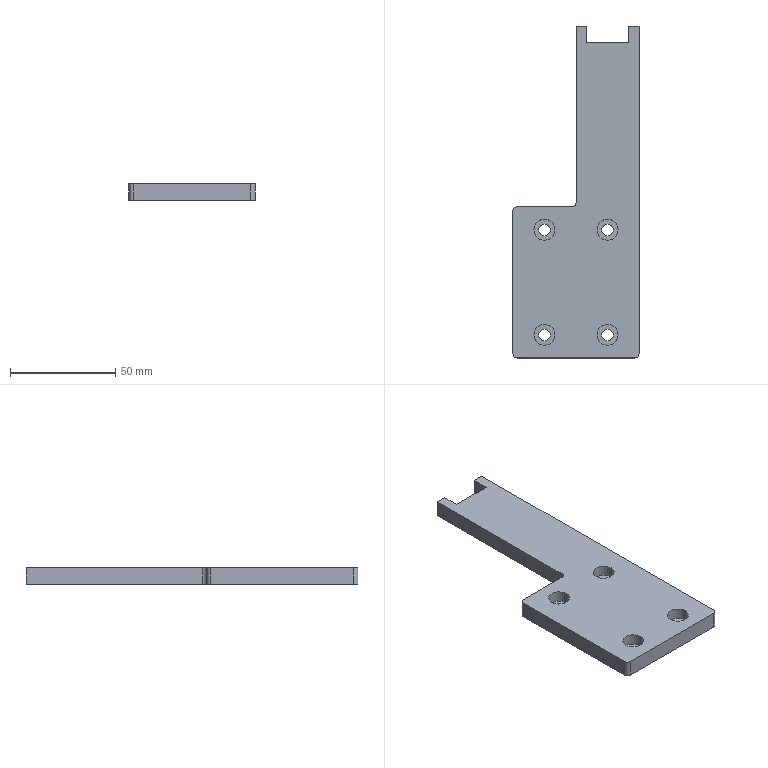Component | SolidWorks | BearingLiftingModule-1_CHEN123-AA-23-1 | 1 solid | 36 faces | box 60 x 158 x 8 mm | volume 51963 mm3 | cylinder 20 | plane 16 | commonest cylinder face diameters 10 x8 5.5 x8 4 x4
build123d program:
from build123d import *

# Parameters (mm, degrees)
SKETCH1_W                                       = 60
SKETCH1_H                                       = 158
BOSS_EXTRUDE1_DEPTH                             = 8
SKETCH2_W                                       = 30
SKETCH2_H                                       = 86
CUT_EXTRUDE1_DEPTH                              = 85.882
SKETCH3_W                                       = 20
SKETCH3_H                                       = 16
CUT_EXTRUDE2_DEPTH                              = 10
FILLET1_R                                       = 2
M5_HEX_SOCKET_HEAD_CAP_SCREW_CBORE1_D           = 5.5
M5_HEX_SOCKET_HEAD_CAP_SCREW_CBORE1_CBORE_D     = 10
M5_HEX_SOCKET_HEAD_CAP_SCREW_CBORE1_CBORE_DEPTH = 5.4


with BuildPart() as part:
    # Sketch1 → Boss-Extrude1 (new body)
    with BuildSketch(Plane.XY):
        Rectangle(SKETCH1_W, SKETCH1_H)
    extrude(amount=BOSS_EXTRUDE1_DEPTH)

    # Sketch2 → Cut-Extrude1 (cut, through all)
    with BuildSketch(Plane.XY.offset(8)):
        with Locations((-15, 36)):
            Rectangle(SKETCH2_W, SKETCH2_H)
    extrude(amount=-CUT_EXTRUDE1_DEPTH, mode=Mode.SUBTRACT)

    # Sketch3 → Cut-Extrude2 (cut)
    with BuildSketch(Plane.XY.offset(8)):
        with Locations((15, 79)):
            Rectangle(SKETCH3_W, SKETCH3_H)
    extrude(amount=-CUT_EXTRUDE2_DEPTH, mode=Mode.SUBTRACT)

    # Fillet1
    fillet1_edges = [part.edges().sort_by_distance(p)[0] for p in [
        (-30, -7, 4),
        (0, -7, 4),
        (30, -79, 4),
        (-30, -79, 4),
    ]]
    fillet(fillet1_edges, radius=FILLET1_R)

    # M5 Hex Socket Head Cap Screw CBORE1 (through all)
    with Locations(Plane.XY.offset(8)):
        with Locations((-15, -18), (15, -18), (-15, -68), (15, -68)):
            CounterBoreHole(M5_HEX_SOCKET_HEAD_CAP_SCREW_CBORE1_D / 2, M5_HEX_SOCKET_HEAD_CAP_SCREW_CBORE1_CBORE_D / 2, M5_HEX_SOCKET_HEAD_CAP_SCREW_CBORE1_CBORE_DEPTH)


solid = part.part

# Placed as in the assembly
solid = solid.moved(Location((54.999, -35.499, 102), (0, 0, 0)))
STEP:
#1=COLOUR_RGB('',0.7922,0.8196,0.9333);
#2=FILL_AREA_STYLE_COLOUR('',#1);
#3=FILL_AREA_STYLE('',(#2));
#4=SURFACE_STYLE_FILL_AREA(#3);
#5=SURFACE_SIDE_STYLE('',(#4));
#6=SURFACE_STYLE_USAGE(.BOTH.,#5);
#7=PRESENTATION_STYLE_ASSIGNMENT((#6));
#8=CARTESIAN_POINT('',(1.378,-2.106,4.118));
#9=VERTEX_POINT('',#8);
#10=CARTESIAN_POINT('',(1.772,-2.106,4.118));
#11=VERTEX_POINT('',#10);
#12=CARTESIAN_POINT('',(1.575,-2.106,4.118));
#13=DIRECTION('',(0.,0.,1.));
#14=DIRECTION('',(1.,0.,0.));
#15=AXIS2_PLACEMENT_3D('',#12,#13,#14);
#16=CIRCLE('',#15,0.1969);
#17=EDGE_CURVE('',#9,#11,#16,.T.);
#18=ORIENTED_EDGE('',*,*,#17,.F.);
#19=CARTESIAN_POINT('',(1.378,-2.106,4.331));
#20=VERTEX_POINT('',#19);
#21=CARTESIAN_POINT('',(1.378,-2.106,4.331));
#22=DIRECTION('',(0.,0.,1.));
#23=VECTOR('',#22,39.37);
#24=LINE('',#21,#23);
#25=EDGE_CURVE('',#9,#20,#24,.T.);
#26=ORIENTED_EDGE('',*,*,#25,.T.);
#27=CARTESIAN_POINT('',(1.772,-2.106,4.331));
#28=VERTEX_POINT('',#27);
#29=CARTESIAN_POINT('',(1.575,-2.106,4.331));
#30=DIRECTION('',(0.,0.,1.));
#31=DIRECTION('',(1.,0.,0.));
#32=AXIS2_PLACEMENT_3D('',#29,#30,#31);
#33=CIRCLE('',#32,0.1969);
#34=EDGE_CURVE('',#20,#28,#33,.T.);
#35=ORIENTED_EDGE('',*,*,#34,.T.);
#36=CARTESIAN_POINT('',(1.772,-2.106,4.331));
#37=DIRECTION('',(0.,0.,1.));
#38=VECTOR('',#37,39.37);
#39=LINE('',#36,#38);
#40=EDGE_CURVE('',#11,#28,#39,.T.);
#41=ORIENTED_EDGE('',*,*,#40,.F.);
#42=EDGE_LOOP('',(#18,#26,#35,#41));
#43=FACE_OUTER_BOUND('',#42,.T.);
#44=CARTESIAN_POINT('',(1.575,-2.106,4.331));
#45=DIRECTION('',(0.,0.,1.));
#46=DIRECTION('',(1.,0.,0.));
#47=AXIS2_PLACEMENT_3D('',#44,#45,#46);
#48=CYLINDRICAL_SURFACE('',#47,0.1969);
#49=ADVANCED_FACE('',(#43),#48,.F.);
#50=CARTESIAN_POINT('',(1.467,-2.106,4.016));
#51=VERTEX_POINT('',#50);
#52=CARTESIAN_POINT('',(1.683,-2.106,4.016));
#53=VERTEX_POINT('',#52);
#54=CARTESIAN_POINT('',(1.575,-2.106,4.016));
#55=DIRECTION('',(0.,0.,1.));
#56=DIRECTION('',(1.,0.,0.));
#57=AXIS2_PLACEMENT_3D('',#54,#55,#56);
#58=CIRCLE('',#57,0.1083);
#59=EDGE_CURVE('',#51,#53,#58,.T.);
#60=ORIENTED_EDGE('',*,*,#59,.F.);
#61=CARTESIAN_POINT('',(1.467,-2.106,4.118));
#62=VERTEX_POINT('',#61);
#63=CARTESIAN_POINT('',(1.467,-2.106,4.331));
#64=DIRECTION('',(0.,0.,1.));
#65=VECTOR('',#64,39.37);
#66=LINE('',#63,#65);
#67=EDGE_CURVE('',#51,#62,#66,.T.);
#68=ORIENTED_EDGE('',*,*,#67,.T.);
#69=CARTESIAN_POINT('',(1.683,-2.106,4.118));
#70=VERTEX_POINT('',#69);
#71=CARTESIAN_POINT('',(1.575,-2.106,4.118));
#72=DIRECTION('',(0.,0.,1.));
#73=DIRECTION('',(1.,0.,0.));
#74=AXIS2_PLACEMENT_3D('',#71,#72,#73);
#75=CIRCLE('',#74,0.1083);
#76=EDGE_CURVE('',#62,#70,#75,.T.);
#77=ORIENTED_EDGE('',*,*,#76,.T.);
#78=CARTESIAN_POINT('',(1.683,-2.106,4.331));
#79=DIRECTION('',(0.,0.,1.));
#80=VECTOR('',#79,39.37);
#81=LINE('',#78,#80);
#82=EDGE_CURVE('',#53,#70,#81,.T.);
#83=ORIENTED_EDGE('',*,*,#82,.F.);
#84=EDGE_LOOP('',(#60,#68,#77,#83));
#85=FACE_OUTER_BOUND('',#84,.T.);
#86=CARTESIAN_POINT('',(1.575,-2.106,4.331));
#87=DIRECTION('',(0.,0.,1.));
#88=DIRECTION('',(1.,0.,0.));
#89=AXIS2_PLACEMENT_3D('',#86,#87,#88);
#90=CYLINDRICAL_SURFACE('',#89,0.1083);
#91=ADVANCED_FACE('',(#85),#90,.F.);
#92=CARTESIAN_POINT('',(2.559,-2.106,4.118));
#93=VERTEX_POINT('',#92);
#94=CARTESIAN_POINT('',(2.953,-2.106,4.118));
#95=VERTEX_POINT('',#94);
#96=CARTESIAN_POINT('',(2.756,-2.106,4.118));
#97=DIRECTION('',(0.,0.,1.));
#98=DIRECTION('',(1.,0.,0.));
#99=AXIS2_PLACEMENT_3D('',#96,#97,#98);
#100=CIRCLE('',#99,0.1969);
#101=EDGE_CURVE('',#93,#95,#100,.T.);
#102=ORIENTED_EDGE('',*,*,#101,.F.);
#103=CARTESIAN_POINT('',(2.559,-2.106,4.331));
#104=VERTEX_POINT('',#103);
#105=CARTESIAN_POINT('',(2.559,-2.106,4.331));
#106=DIRECTION('',(0.,0.,1.));
#107=VECTOR('',#106,39.37);
#108=LINE('',#105,#107);
#109=EDGE_CURVE('',#93,#104,#108,.T.);
#110=ORIENTED_EDGE('',*,*,#109,.T.);
#111=CARTESIAN_POINT('',(2.953,-2.106,4.331));
#112=VERTEX_POINT('',#111);
#113=CARTESIAN_POINT('',(2.756,-2.106,4.331));
#114=DIRECTION('',(0.,0.,1.));
#115=DIRECTION('',(1.,0.,0.));
#116=AXIS2_PLACEMENT_3D('',#113,#114,#115);
#117=CIRCLE('',#116,0.1969);
#118=EDGE_CURVE('',#104,#112,#117,.T.);
#119=ORIENTED_EDGE('',*,*,#118,.T.);
#120=CARTESIAN_POINT('',(2.953,-2.106,4.331));
#121=DIRECTION('',(0.,0.,1.));
#122=VECTOR('',#121,39.37);
#123=LINE('',#120,#122);
#124=EDGE_CURVE('',#95,#112,#123,.T.);
#125=ORIENTED_EDGE('',*,*,#124,.F.);
#126=EDGE_LOOP('',(#102,#110,#119,#125));
#127=FACE_OUTER_BOUND('',#126,.T.);
#128=CARTESIAN_POINT('',(2.756,-2.106,4.331));
#129=DIRECTION('',(0.,0.,1.));
#130=DIRECTION('',(1.,0.,0.));
#131=AXIS2_PLACEMENT_3D('',#128,#129,#130);
#132=CYLINDRICAL_SURFACE('',#131,0.1969);
#133=ADVANCED_FACE('',(#127),#132,.F.);
#134=CARTESIAN_POINT('',(2.648,-2.106,4.016));
#135=VERTEX_POINT('',#134);
#136=CARTESIAN_POINT('',(2.864,-2.106,4.016));
#137=VERTEX_POINT('',#136);
#138=CARTESIAN_POINT('',(2.756,-2.106,4.016));
#139=DIRECTION('',(0.,0.,1.));
#140=DIRECTION('',(1.,0.,0.));
#141=AXIS2_PLACEMENT_3D('',#138,#139,#140);
#142=CIRCLE('',#141,0.1083);
#143=EDGE_CURVE('',#135,#137,#142,.T.);
#144=ORIENTED_EDGE('',*,*,#143,.F.);
#145=CARTESIAN_POINT('',(2.648,-2.106,4.118));
#146=VERTEX_POINT('',#145);
#147=CARTESIAN_POINT('',(2.648,-2.106,4.331));
#148=DIRECTION('',(0.,0.,1.));
#149=VECTOR('',#148,39.37);
#150=LINE('',#147,#149);
#151=EDGE_CURVE('',#135,#146,#150,.T.);
#152=ORIENTED_EDGE('',*,*,#151,.T.);
#153=CARTESIAN_POINT('',(2.864,-2.106,4.118));
#154=VERTEX_POINT('',#153);
#155=CARTESIAN_POINT('',(2.756,-2.106,4.118));
#156=DIRECTION('',(0.,0.,1.));
#157=DIRECTION('',(1.,0.,0.));
#158=AXIS2_PLACEMENT_3D('',#155,#156,#157);
#159=CIRCLE('',#158,0.1083);
#160=EDGE_CURVE('',#146,#154,#159,.T.);
#161=ORIENTED_EDGE('',*,*,#160,.T.);
#162=CARTESIAN_POINT('',(2.864,-2.106,4.331));
#163=DIRECTION('',(0.,0.,1.));
#164=VECTOR('',#163,39.37);
#165=LINE('',#162,#164);
#166=EDGE_CURVE('',#137,#154,#165,.T.);
#167=ORIENTED_EDGE('',*,*,#166,.F.);
#168=EDGE_LOOP('',(#144,#152,#161,#167));
#169=FACE_OUTER_BOUND('',#168,.T.);
#170=CARTESIAN_POINT('',(2.756,-2.106,4.331));
#171=DIRECTION('',(0.,0.,1.));
#172=DIRECTION('',(1.,0.,0.));
#173=AXIS2_PLACEMENT_3D('',#170,#171,#172);
#174=CYLINDRICAL_SURFACE('',#173,0.1083);
#175=ADVANCED_FACE('',(#169),#174,.F.);
#176=CARTESIAN_POINT('',(1.378,-4.075,4.118));
#177=VERTEX_POINT('',#176);
#178=CARTESIAN_POINT('',(1.772,-4.075,4.118));
#179=VERTEX_POINT('',#178);
#180=CARTESIAN_POINT('',(1.575,-4.075,4.118));
#181=DIRECTION('',(0.,0.,1.));
#182=DIRECTION('',(1.,0.,0.));
#183=AXIS2_PLACEMENT_3D('',#180,#181,#182);
#184=CIRCLE('',#183,0.1969);
#185=EDGE_CURVE('',#177,#179,#184,.T.);
#186=ORIENTED_EDGE('',*,*,#185,.F.);
#187=CARTESIAN_POINT('',(1.378,-4.075,4.331));
#188=VERTEX_POINT('',#187);
#189=CARTESIAN_POINT('',(1.378,-4.075,4.331));
#190=DIRECTION('',(0.,0.,1.));
#191=VECTOR('',#190,39.37);
#192=LINE('',#189,#191);
#193=EDGE_CURVE('',#177,#188,#192,.T.);
#194=ORIENTED_EDGE('',*,*,#193,.T.);
#195=CARTESIAN_POINT('',(1.772,-4.075,4.331));
#196=VERTEX_POINT('',#195);
#197=CARTESIAN_POINT('',(1.575,-4.075,4.331));
#198=DIRECTION('',(0.,0.,1.));
#199=DIRECTION('',(1.,0.,0.));
#200=AXIS2_PLACEMENT_3D('',#197,#198,#199);
#201=CIRCLE('',#200,0.1969);
#202=EDGE_CURVE('',#188,#196,#201,.T.);
#203=ORIENTED_EDGE('',*,*,#202,.T.);
#204=CARTESIAN_POINT('',(1.772,-4.075,4.331));
#205=DIRECTION('',(0.,0.,1.));
#206=VECTOR('',#205,39.37);
#207=LINE('',#204,#206);
#208=EDGE_CURVE('',#179,#196,#207,.T.);
#209=ORIENTED_EDGE('',*,*,#208,.F.);
#210=EDGE_LOOP('',(#186,#194,#203,#209));
#211=FACE_OUTER_BOUND('',#210,.T.);
#212=CARTESIAN_POINT('',(1.575,-4.075,4.331));
#213=DIRECTION('',(0.,0.,1.));
#214=DIRECTION('',(1.,0.,0.));
#215=AXIS2_PLACEMENT_3D('',#212,#213,#214);
#216=CYLINDRICAL_SURFACE('',#215,0.1969);
#217=ADVANCED_FACE('',(#211),#216,.F.);
#218=CARTESIAN_POINT('',(1.467,-4.075,4.016));
#219=VERTEX_POINT('',#218);
#220=CARTESIAN_POINT('',(1.683,-4.075,4.016));
#221=VERTEX_POINT('',#220);
#222=CARTESIAN_POINT('',(1.575,-4.075,4.016));
#223=DIRECTION('',(0.,0.,1.));
#224=DIRECTION('',(1.,0.,0.));
#225=AXIS2_PLACEMENT_3D('',#222,#223,#224);
#226=CIRCLE('',#225,0.1083);
#227=EDGE_CURVE('',#219,#221,#226,.T.);
#228=ORIENTED_EDGE('',*,*,#227,.F.);
#229=CARTESIAN_POINT('',(1.467,-4.075,4.118));
#230=VERTEX_POINT('',#229);
#231=CARTESIAN_POINT('',(1.467,-4.075,4.331));
#232=DIRECTION('',(0.,0.,1.));
#233=VECTOR('',#232,39.37);
#234=LINE('',#231,#233);
#235=EDGE_CURVE('',#219,#230,#234,.T.);
#236=ORIENTED_EDGE('',*,*,#235,.T.);
#237=CARTESIAN_POINT('',(1.683,-4.075,4.118));
#238=VERTEX_POINT('',#237);
#239=CARTESIAN_POINT('',(1.575,-4.075,4.118));
#240=DIRECTION('',(0.,0.,1.));
#241=DIRECTION('',(1.,0.,0.));
#242=AXIS2_PLACEMENT_3D('',#239,#240,#241);
#243=CIRCLE('',#242,0.1083);
#244=EDGE_CURVE('',#230,#238,#243,.T.);
#245=ORIENTED_EDGE('',*,*,#244,.T.);
#246=CARTESIAN_POINT('',(1.683,-4.075,4.331));
#247=DIRECTION('',(0.,0.,1.));
#248=VECTOR('',#247,39.37);
#249=LINE('',#246,#248);
#250=EDGE_CURVE('',#221,#238,#249,.T.);
#251=ORIENTED_EDGE('',*,*,#250,.F.);
#252=EDGE_LOOP('',(#228,#236,#245,#251));
#253=FACE_OUTER_BOUND('',#252,.T.);
#254=CARTESIAN_POINT('',(1.575,-4.075,4.331));
#255=DIRECTION('',(0.,0.,1.));
#256=DIRECTION('',(1.,0.,0.));
#257=AXIS2_PLACEMENT_3D('',#254,#255,#256);
#258=CYLINDRICAL_SURFACE('',#257,0.1083);
#259=ADVANCED_FACE('',(#253),#258,.F.);
#260=CARTESIAN_POINT('',(2.559,-4.075,4.118));
#261=VERTEX_POINT('',#260);
#262=CARTESIAN_POINT('',(2.953,-4.075,4.118));
#263=VERTEX_POINT('',#262);
#264=CARTESIAN_POINT('',(2.756,-4.075,4.118));
#265=DIRECTION('',(0.,0.,1.));
#266=DIRECTION('',(1.,0.,0.));
#267=AXIS2_PLACEMENT_3D('',#264,#265,#266);
#268=CIRCLE('',#267,0.1969);
#269=EDGE_CURVE('',#261,#263,#268,.T.);
#270=ORIENTED_EDGE('',*,*,#269,.F.);
#271=CARTESIAN_POINT('',(2.559,-4.075,4.331));
#272=VERTEX_POINT('',#271);
#273=CARTESIAN_POINT('',(2.559,-4.075,4.331));
#274=DIRECTION('',(0.,0.,1.));
#275=VECTOR('',#274,39.37);
#276=LINE('',#273,#275);
#277=EDGE_CURVE('',#261,#272,#276,.T.);
#278=ORIENTED_EDGE('',*,*,#277,.T.);
#279=CARTESIAN_POINT('',(2.953,-4.075,4.331));
#280=VERTEX_POINT('',#279);
#281=CARTESIAN_POINT('',(2.756,-4.075,4.331));
#282=DIRECTION('',(0.,0.,1.));
#283=DIRECTION('',(1.,0.,0.));
#284=AXIS2_PLACEMENT_3D('',#281,#282,#283);
#285=CIRCLE('',#284,0.1969);
#286=EDGE_CURVE('',#272,#280,#285,.T.);
#287=ORIENTED_EDGE('',*,*,#286,.T.);
#288=CARTESIAN_POINT('',(2.953,-4.075,4.331));
#289=DIRECTION('',(0.,0.,1.));
#290=VECTOR('',#289,39.37);
#291=LINE('',#288,#290);
#292=EDGE_CURVE('',#263,#280,#291,.T.);
#293=ORIENTED_EDGE('',*,*,#292,.F.);
#294=EDGE_LOOP('',(#270,#278,#287,#293));
#295=FACE_OUTER_BOUND('',#294,.T.);
#296=CARTESIAN_POINT('',(2.756,-4.075,4.331));
#297=DIRECTION('',(0.,0.,1.));
#298=DIRECTION('',(1.,0.,0.));
#299=AXIS2_PLACEMENT_3D('',#296,#297,#298);
#300=CYLINDRICAL_SURFACE('',#299,0.1969);
#301=ADVANCED_FACE('',(#295),#300,.F.);
#302=CARTESIAN_POINT('',(2.648,-4.075,4.016));
#303=VERTEX_POINT('',#302);
#304=CARTESIAN_POINT('',(2.864,-4.075,4.016));
#305=VERTEX_POINT('',#304);
#306=CARTESIAN_POINT('',(2.756,-4.075,4.016));
#307=DIRECTION('',(0.,0.,1.));
#308=DIRECTION('',(1.,0.,0.));
#309=AXIS2_PLACEMENT_3D('',#306,#307,#308);
#310=CIRCLE('',#309,0.1083);
#311=EDGE_CURVE('',#303,#305,#310,.T.);
#312=ORIENTED_EDGE('',*,*,#311,.F.);
#313=CARTESIAN_POINT('',(2.648,-4.075,4.118));
#314=VERTEX_POINT('',#313);
#315=CARTESIAN_POINT('',(2.648,-4.075,4.331));
#316=DIRECTION('',(0.,0.,1.));
#317=VECTOR('',#316,39.37);
#318=LINE('',#315,#317);
#319=EDGE_CURVE('',#303,#314,#318,.T.);
#320=ORIENTED_EDGE('',*,*,#319,.T.);
#321=CARTESIAN_POINT('',(2.864,-4.075,4.118));
#322=VERTEX_POINT('',#321);
#323=CARTESIAN_POINT('',(2.756,-4.075,4.118));
#324=DIRECTION('',(0.,0.,1.));
#325=DIRECTION('',(1.,0.,0.));
#326=AXIS2_PLACEMENT_3D('',#323,#324,#325);
#327=CIRCLE('',#326,0.1083);
#328=EDGE_CURVE('',#314,#322,#327,.T.);
#329=ORIENTED_EDGE('',*,*,#328,.T.);
#330=CARTESIAN_POINT('',(2.864,-4.075,4.331));
#331=DIRECTION('',(0.,0.,1.));
#332=VECTOR('',#331,39.37);
#333=LINE('',#330,#332);
#334=EDGE_CURVE('',#305,#322,#333,.T.);
#335=ORIENTED_EDGE('',*,*,#334,.F.);
#336=EDGE_LOOP('',(#312,#320,#329,#335));
#337=FACE_OUTER_BOUND('',#336,.T.);
#338=CARTESIAN_POINT('',(2.756,-4.075,4.331));
#339=DIRECTION('',(0.,0.,1.));
#340=DIRECTION('',(1.,0.,0.));
#341=AXIS2_PLACEMENT_3D('',#338,#339,#340);
#342=CYLINDRICAL_SURFACE('',#341,0.1083);
#343=ADVANCED_FACE('',(#337),#342,.F.);
#344=CARTESIAN_POINT('',(3.346,1.713,4.016));
#345=VERTEX_POINT('',#344);
#346=CARTESIAN_POINT('',(3.15,1.713,4.016));
#347=VERTEX_POINT('',#346);
#348=CARTESIAN_POINT('',(0.9842,1.713,4.016));
#349=DIRECTION('',(-1.,0.,0.));
#350=VECTOR('',#349,39.37);
#351=LINE('',#348,#350);
#352=EDGE_CURVE('',#345,#347,#351,.T.);
#353=ORIENTED_EDGE('',*,*,#352,.T.);
#354=CARTESIAN_POINT('',(3.15,1.713,4.331));
#355=VERTEX_POINT('',#354);
#356=CARTESIAN_POINT('',(3.15,1.713,4.331));
#357=DIRECTION('',(0.,0.,1.));
#358=VECTOR('',#357,39.37);
#359=LINE('',#356,#358);
#360=EDGE_CURVE('',#347,#355,#359,.T.);
#361=ORIENTED_EDGE('',*,*,#360,.T.);
#362=CARTESIAN_POINT('',(3.346,1.713,4.331));
#363=VERTEX_POINT('',#362);
#364=CARTESIAN_POINT('',(0.9842,1.713,4.331));
#365=DIRECTION('',(-1.,0.,0.));
#366=VECTOR('',#365,39.37);
#367=LINE('',#364,#366);
#368=EDGE_CURVE('',#363,#355,#367,.T.);
#369=ORIENTED_EDGE('',*,*,#368,.F.);
#370=CARTESIAN_POINT('',(3.346,1.713,4.331));
#371=DIRECTION('',(0.,0.,-1.));
#372=VECTOR('',#371,39.37);
#373=LINE('',#370,#372);
#374=EDGE_CURVE('',#363,#345,#373,.T.);
#375=ORIENTED_EDGE('',*,*,#374,.T.);
#376=EDGE_LOOP('',(#353,#361,#369,#375));
#377=FACE_OUTER_BOUND('',#376,.T.);
#378=CARTESIAN_POINT('',(0.9842,1.713,4.331));
#379=DIRECTION('',(0.,-1.,0.));
#380=DIRECTION('',(0.,0.,-1.));
#381=AXIS2_PLACEMENT_3D('',#378,#379,#380);
#382=PLANE('',#381);
#383=ADVANCED_FACE('',(#377),#382,.F.);
#384=CARTESIAN_POINT('',(3.346,-4.429,4.331));
#385=VERTEX_POINT('',#384);
#386=CARTESIAN_POINT('',(3.346,-4.508,4.331));
#387=DIRECTION('',(0.,1.,0.));
#388=VECTOR('',#387,39.37);
#389=LINE('',#386,#388);
#390=EDGE_CURVE('',#385,#363,#389,.T.);
#391=ORIENTED_EDGE('',*,*,#390,.F.);
#392=CARTESIAN_POINT('',(3.346,-4.429,4.016));
#393=VERTEX_POINT('',#392);
#394=CARTESIAN_POINT('',(3.346,-4.429,4.331));
#395=DIRECTION('',(0.,0.,-1.));
#396=VECTOR('',#395,39.37);
#397=LINE('',#394,#396);
#398=EDGE_CURVE('',#385,#393,#397,.T.);
#399=ORIENTED_EDGE('',*,*,#398,.T.);
#400=CARTESIAN_POINT('',(3.346,-4.508,4.016));
#401=DIRECTION('',(0.,1.,0.));
#402=VECTOR('',#401,39.37);
#403=LINE('',#400,#402);
#404=EDGE_CURVE('',#393,#345,#403,.T.);
#405=ORIENTED_EDGE('',*,*,#404,.T.);
#406=ORIENTED_EDGE('',*,*,#374,.F.);
#407=EDGE_LOOP('',(#391,#399,#405,#406));
#408=FACE_OUTER_BOUND('',#407,.T.);
#409=CARTESIAN_POINT('',(3.346,-4.508,4.331));
#410=DIRECTION('',(-1.,0.,0.));
#411=DIRECTION('',(0.,0.,1.));
#412=AXIS2_PLACEMENT_3D('',#409,#410,#411);
#413=PLANE('',#412);
#414=ADVANCED_FACE('',(#408),#413,.F.);
#415=CARTESIAN_POINT('',(2.362,1.713,4.331));
#416=VERTEX_POINT('',#415);
#417=CARTESIAN_POINT('',(2.165,1.713,4.331));
#418=VERTEX_POINT('',#417);
#419=CARTESIAN_POINT('',(0.9842,1.713,4.331));
#420=DIRECTION('',(-1.,0.,0.));
#421=VECTOR('',#420,39.37);
#422=LINE('',#419,#421);
#423=EDGE_CURVE('',#416,#418,#422,.T.);
#424=ORIENTED_EDGE('',*,*,#423,.F.);
#425=CARTESIAN_POINT('',(2.362,1.713,4.016));
#426=VERTEX_POINT('',#425);
#427=CARTESIAN_POINT('',(2.362,1.713,4.331));
#428=DIRECTION('',(0.,0.,-1.));
#429=VECTOR('',#428,39.37);
#430=LINE('',#427,#429);
#431=EDGE_CURVE('',#416,#426,#430,.T.);
#432=ORIENTED_EDGE('',*,*,#431,.T.);
#433=CARTESIAN_POINT('',(2.165,1.713,4.016));
#434=VERTEX_POINT('',#433);
#435=CARTESIAN_POINT('',(0.9842,1.713,4.016));
#436=DIRECTION('',(-1.,0.,0.));
#437=VECTOR('',#436,39.37);
#438=LINE('',#435,#437);
#439=EDGE_CURVE('',#426,#434,#438,.T.);
#440=ORIENTED_EDGE('',*,*,#439,.T.);
#441=CARTESIAN_POINT('',(2.165,1.713,4.016));
#442=DIRECTION('',(0.,0.,1.));
#443=VECTOR('',#442,39.37);
#444=LINE('',#441,#443);
#445=EDGE_CURVE('',#434,#418,#444,.T.);
#446=ORIENTED_EDGE('',*,*,#445,.T.);
#447=EDGE_LOOP('',(#424,#432,#440,#446));
#448=FACE_OUTER_BOUND('',#447,.T.);
#449=CARTESIAN_POINT('',(0.9842,1.713,4.331));
#450=DIRECTION('',(0.,-1.,0.));
#451=DIRECTION('',(0.,0.,-1.));
#452=AXIS2_PLACEMENT_3D('',#449,#450,#451);
#453=PLANE('',#452);
#454=ADVANCED_FACE('',(#448),#453,.F.);
#455=CARTESIAN_POINT('',(0.9842,-1.752,4.016));
#456=VERTEX_POINT('',#455);
#457=CARTESIAN_POINT('',(0.9842,-4.429,4.016));
#458=VERTEX_POINT('',#457);
#459=CARTESIAN_POINT('',(0.9842,-4.508,4.016));
#460=DIRECTION('',(0.,-1.,0.));
#461=VECTOR('',#460,39.37);
#462=LINE('',#459,#461);
#463=EDGE_CURVE('',#456,#458,#462,.T.);
#464=ORIENTED_EDGE('',*,*,#463,.T.);
#465=CARTESIAN_POINT('',(0.9842,-4.429,4.331));
#466=VERTEX_POINT('',#465);
#467=CARTESIAN_POINT('',(0.9842,-4.429,4.331));
#468=DIRECTION('',(0.,0.,1.));
#469=VECTOR('',#468,39.37);
#470=LINE('',#467,#469);
#471=EDGE_CURVE('',#458,#466,#470,.T.);
#472=ORIENTED_EDGE('',*,*,#471,.T.);
#473=CARTESIAN_POINT('',(0.9842,-1.752,4.331));
#474=VERTEX_POINT('',#473);
#475=CARTESIAN_POINT('',(0.9842,-4.508,4.331));
#476=DIRECTION('',(0.,-1.,0.));
#477=VECTOR('',#476,39.37);
#478=LINE('',#475,#477);
#479=EDGE_CURVE('',#474,#466,#478,.T.);
#480=ORIENTED_EDGE('',*,*,#479,.F.);
#481=CARTESIAN_POINT('',(0.9842,-1.752,4.331));
#482=DIRECTION('',(0.,0.,-1.));
#483=VECTOR('',#482,39.37);
#484=LINE('',#481,#483);
#485=EDGE_CURVE('',#474,#456,#484,.T.);
#486=ORIENTED_EDGE('',*,*,#485,.T.);
#487=EDGE_LOOP('',(#464,#472,#480,#486));
#488=FACE_OUTER_BOUND('',#487,.T.);
#489=CARTESIAN_POINT('',(0.9842,-4.508,4.331));
#490=DIRECTION('',(1.,0.,0.));
#491=DIRECTION('',(0.,0.,-1.));
#492=AXIS2_PLACEMENT_3D('',#489,#490,#491);
#493=PLANE('',#492);
#494=ADVANCED_FACE('',(#488),#493,.F.);
#495=CARTESIAN_POINT('',(1.063,-4.508,4.016));
#496=VERTEX_POINT('',#495);
#497=CARTESIAN_POINT('',(3.268,-4.508,4.016));
#498=VERTEX_POINT('',#497);
#499=CARTESIAN_POINT('',(0.9842,-4.508,4.016));
#500=DIRECTION('',(1.,0.,0.));
#501=VECTOR('',#500,39.37);
#502=LINE('',#499,#501);
#503=EDGE_CURVE('',#496,#498,#502,.T.);
#504=ORIENTED_EDGE('',*,*,#503,.T.);
#505=CARTESIAN_POINT('',(3.268,-4.508,4.331));
#506=VERTEX_POINT('',#505);
#507=CARTESIAN_POINT('',(3.268,-4.508,4.331));
#508=DIRECTION('',(0.,0.,1.));
#509=VECTOR('',#508,39.37);
#510=LINE('',#507,#509);
#511=EDGE_CURVE('',#498,#506,#510,.T.);
#512=ORIENTED_EDGE('',*,*,#511,.T.);
#513=CARTESIAN_POINT('',(1.063,-4.508,4.331));
#514=VERTEX_POINT('',#513);
#515=CARTESIAN_POINT('',(0.9842,-4.508,4.331));
#516=DIRECTION('',(1.,0.,0.));
#517=VECTOR('',#516,39.37);
#518=LINE('',#515,#517);
#519=EDGE_CURVE('',#514,#506,#518,.T.);
#520=ORIENTED_EDGE('',*,*,#519,.F.);
#521=CARTESIAN_POINT('',(1.063,-4.508,4.331));
#522=DIRECTION('',(0.,0.,-1.));
#523=VECTOR('',#522,39.37);
#524=LINE('',#521,#523);
#525=EDGE_CURVE('',#514,#496,#524,.T.);
#526=ORIENTED_EDGE('',*,*,#525,.T.);
#527=EDGE_LOOP('',(#504,#512,#520,#526));
#528=FACE_OUTER_BOUND('',#527,.T.);
#529=CARTESIAN_POINT('',(0.9842,-4.508,4.331));
#530=DIRECTION('',(0.,1.,0.));
#531=DIRECTION('',(0.,0.,1.));
#532=AXIS2_PLACEMENT_3D('',#529,#530,#531);
#533=PLANE('',#532);
#534=ADVANCED_FACE('',(#528),#533,.F.);
#535=CARTESIAN_POINT('',(1.575,-2.106,4.331));
#536=DIRECTION('',(0.,0.,1.));
#537=DIRECTION('',(1.,0.,0.));
#538=AXIS2_PLACEMENT_3D('',#535,#536,#537);
#539=CIRCLE('',#538,0.1969);
#540=EDGE_CURVE('',#28,#20,#539,.T.);
#541=ORIENTED_EDGE('',*,*,#540,.F.);
#542=ORIENTED_EDGE('',*,*,#34,.F.);
#543=EDGE_LOOP('',(#541,#542));
#544=FACE_BOUND('',#543,.T.);
#545=CARTESIAN_POINT('',(2.756,-2.106,4.331));
#546=DIRECTION('',(0.,0.,1.));
#547=DIRECTION('',(1.,0.,0.));
#548=AXIS2_PLACEMENT_3D('',#545,#546,#547);
#549=CIRCLE('',#548,0.1969);
#550=EDGE_CURVE('',#112,#104,#549,.T.);
#551=ORIENTED_EDGE('',*,*,#550,.F.);
#552=ORIENTED_EDGE('',*,*,#118,.F.);
#553=EDGE_LOOP('',(#551,#552));
#554=FACE_BOUND('',#553,.T.);
#555=CARTESIAN_POINT('',(1.575,-4.075,4.331));
#556=DIRECTION('',(0.,0.,1.));
#557=DIRECTION('',(1.,0.,0.));
#558=AXIS2_PLACEMENT_3D('',#555,#556,#557);
#559=CIRCLE('',#558,0.1969);
#560=EDGE_CURVE('',#196,#188,#559,.T.);
#561=ORIENTED_EDGE('',*,*,#560,.F.);
#562=ORIENTED_EDGE('',*,*,#202,.F.);
#563=EDGE_LOOP('',(#561,#562));
#564=FACE_BOUND('',#563,.T.);
#565=CARTESIAN_POINT('',(2.756,-4.075,4.331));
#566=DIRECTION('',(0.,0.,1.));
#567=DIRECTION('',(1.,0.,0.));
#568=AXIS2_PLACEMENT_3D('',#565,#566,#567);
#569=CIRCLE('',#568,0.1969);
#570=EDGE_CURVE('',#280,#272,#569,.T.);
#571=ORIENTED_EDGE('',*,*,#570,.F.);
#572=ORIENTED_EDGE('',*,*,#286,.F.);
#573=EDGE_LOOP('',(#571,#572));
#574=FACE_BOUND('',#573,.T.);
#575=ORIENTED_EDGE('',*,*,#519,.T.);
#576=CARTESIAN_POINT('',(3.268,-4.429,4.331));
#577=DIRECTION('',(0.,0.,1.));
#578=DIRECTION('',(-1.,0.,0.));
#579=AXIS2_PLACEMENT_3D('',#576,#577,#578);
#580=CIRCLE('',#579,0.07874);
#581=EDGE_CURVE('',#506,#385,#580,.T.);
#582=ORIENTED_EDGE('',*,*,#581,.T.);
#583=ORIENTED_EDGE('',*,*,#390,.T.);
#584=ORIENTED_EDGE('',*,*,#368,.T.);
#585=CARTESIAN_POINT('',(3.15,1.398,4.331));
#586=VERTEX_POINT('',#585);
#587=CARTESIAN_POINT('',(3.15,1.398,4.331));
#588=DIRECTION('',(0.,1.,0.));
#589=VECTOR('',#588,39.37);
#590=LINE('',#587,#589);
#591=EDGE_CURVE('',#586,#355,#590,.T.);
#592=ORIENTED_EDGE('',*,*,#591,.F.);
#593=CARTESIAN_POINT('',(2.362,1.398,4.331));
#594=VERTEX_POINT('',#593);
#595=CARTESIAN_POINT('',(2.362,1.398,4.331));
#596=DIRECTION('',(1.,0.,0.));
#597=VECTOR('',#596,39.37);
#598=LINE('',#595,#597);
#599=EDGE_CURVE('',#594,#586,#598,.T.);
#600=ORIENTED_EDGE('',*,*,#599,.F.);
#601=CARTESIAN_POINT('',(2.362,1.398,4.331));
#602=DIRECTION('',(0.,-1.,0.));
#603=VECTOR('',#602,39.37);
#604=LINE('',#601,#603);
#605=EDGE_CURVE('',#416,#594,#604,.T.);
#606=ORIENTED_EDGE('',*,*,#605,.F.);
#607=ORIENTED_EDGE('',*,*,#423,.T.);
#608=CARTESIAN_POINT('',(2.165,-1.594,4.331));
#609=VERTEX_POINT('',#608);
#610=CARTESIAN_POINT('',(2.165,1.713,4.331));
#611=DIRECTION('',(-0.,1.,0.));
#612=VECTOR('',#611,39.37);
#613=LINE('',#610,#612);
#614=EDGE_CURVE('',#609,#418,#613,.T.);
#615=ORIENTED_EDGE('',*,*,#614,.F.);
#616=CARTESIAN_POINT('',(2.087,-1.673,4.331));
#617=VERTEX_POINT('',#616);
#618=CARTESIAN_POINT('',(2.087,-1.594,4.331));
#619=DIRECTION('',(0.,0.,-1.));
#620=DIRECTION('',(-1.,0.,0.));
#621=AXIS2_PLACEMENT_3D('',#618,#619,#620);
#622=CIRCLE('',#621,0.07874);
#623=EDGE_CURVE('',#609,#617,#622,.T.);
#624=ORIENTED_EDGE('',*,*,#623,.T.);
#625=CARTESIAN_POINT('',(1.063,-1.673,4.331));
#626=VERTEX_POINT('',#625);
#627=CARTESIAN_POINT('',(0.9842,-1.673,4.331));
#628=DIRECTION('',(1.,0.,0.));
#629=VECTOR('',#628,39.37);
#630=LINE('',#627,#629);
#631=EDGE_CURVE('',#626,#617,#630,.T.);
#632=ORIENTED_EDGE('',*,*,#631,.F.);
#633=CARTESIAN_POINT('',(1.063,-1.752,4.331));
#634=DIRECTION('',(0.,0.,1.));
#635=DIRECTION('',(-1.,0.,0.));
#636=AXIS2_PLACEMENT_3D('',#633,#634,#635);
#637=CIRCLE('',#636,0.07874);
#638=EDGE_CURVE('',#626,#474,#637,.T.);
#639=ORIENTED_EDGE('',*,*,#638,.T.);
#640=ORIENTED_EDGE('',*,*,#479,.T.);
#641=CARTESIAN_POINT('',(1.063,-4.429,4.331));
#642=DIRECTION('',(0.,0.,1.));
#643=DIRECTION('',(-1.,0.,0.));
#644=AXIS2_PLACEMENT_3D('',#641,#642,#643);
#645=CIRCLE('',#644,0.07874);
#646=EDGE_CURVE('',#466,#514,#645,.T.);
#647=ORIENTED_EDGE('',*,*,#646,.T.);
#648=EDGE_LOOP('',(#575,#582,#583,#584,#592,#600,#606,#607,#615,#624,#632,#639,#640,#647));
#649=FACE_OUTER_BOUND('',#648,.T.);
#650=CARTESIAN_POINT('',(2.165,-1.398,4.331));
#651=DIRECTION('',(0.,0.,-1.));
#652=DIRECTION('',(-1.,0.,0.));
#653=AXIS2_PLACEMENT_3D('',#650,#651,#652);
#654=PLANE('',#653);
#655=ADVANCED_FACE('',(#544,#554,#564,#574,#649),#654,.F.);
#656=CARTESIAN_POINT('',(1.575,-2.106,4.016));
#657=DIRECTION('',(0.,0.,1.));
#658=DIRECTION('',(1.,0.,0.));
#659=AXIS2_PLACEMENT_3D('',#656,#657,#658);
#660=CIRCLE('',#659,0.1083);
#661=EDGE_CURVE('',#53,#51,#660,.T.);
#662=ORIENTED_EDGE('',*,*,#661,.T.);
#663=ORIENTED_EDGE('',*,*,#59,.T.);
#664=EDGE_LOOP('',(#662,#663));
#665=FACE_BOUND('',#664,.T.);
#666=CARTESIAN_POINT('',(2.756,-2.106,4.016));
#667=DIRECTION('',(0.,0.,1.));
#668=DIRECTION('',(1.,0.,0.));
#669=AXIS2_PLACEMENT_3D('',#666,#667,#668);
#670=CIRCLE('',#669,0.1083);
#671=EDGE_CURVE('',#137,#135,#670,.T.);
#672=ORIENTED_EDGE('',*,*,#671,.T.);
#673=ORIENTED_EDGE('',*,*,#143,.T.);
#674=EDGE_LOOP('',(#672,#673));
#675=FACE_BOUND('',#674,.T.);
#676=CARTESIAN_POINT('',(1.575,-4.075,4.016));
#677=DIRECTION('',(0.,0.,1.));
#678=DIRECTION('',(1.,0.,0.));
#679=AXIS2_PLACEMENT_3D('',#676,#677,#678);
#680=CIRCLE('',#679,0.1083);
#681=EDGE_CURVE('',#221,#219,#680,.T.);
#682=ORIENTED_EDGE('',*,*,#681,.T.);
#683=ORIENTED_EDGE('',*,*,#227,.T.);
#684=EDGE_LOOP('',(#682,#683));
#685=FACE_BOUND('',#684,.T.);
#686=CARTESIAN_POINT('',(2.756,-4.075,4.016));
#687=DIRECTION('',(0.,0.,1.));
#688=DIRECTION('',(1.,0.,0.));
#689=AXIS2_PLACEMENT_3D('',#686,#687,#688);
#690=CIRCLE('',#689,0.1083);
#691=EDGE_CURVE('',#305,#303,#690,.T.);
#692=ORIENTED_EDGE('',*,*,#691,.T.);
#693=ORIENTED_EDGE('',*,*,#311,.T.);
#694=EDGE_LOOP('',(#692,#693));
#695=FACE_BOUND('',#694,.T.);
#696=ORIENTED_EDGE('',*,*,#404,.F.);
#697=CARTESIAN_POINT('',(3.268,-4.429,4.016));
#698=DIRECTION('',(0.,0.,-1.));
#699=DIRECTION('',(-1.,0.,0.));
#700=AXIS2_PLACEMENT_3D('',#697,#698,#699);
#701=CIRCLE('',#700,0.07874);
#702=EDGE_CURVE('',#393,#498,#701,.T.);
#703=ORIENTED_EDGE('',*,*,#702,.T.);
#704=ORIENTED_EDGE('',*,*,#503,.F.);
#705=CARTESIAN_POINT('',(1.063,-4.429,4.016));
#706=DIRECTION('',(0.,0.,-1.));
#707=DIRECTION('',(-1.,0.,0.));
#708=AXIS2_PLACEMENT_3D('',#705,#706,#707);
#709=CIRCLE('',#708,0.07874);
#710=EDGE_CURVE('',#496,#458,#709,.T.);
#711=ORIENTED_EDGE('',*,*,#710,.T.);
#712=ORIENTED_EDGE('',*,*,#463,.F.);
#713=CARTESIAN_POINT('',(1.063,-1.673,4.016));
#714=VERTEX_POINT('',#713);
#715=CARTESIAN_POINT('',(1.063,-1.752,4.016));
#716=DIRECTION('',(0.,0.,-1.));
#717=DIRECTION('',(-1.,0.,0.));
#718=AXIS2_PLACEMENT_3D('',#715,#716,#717);
#719=CIRCLE('',#718,0.07874);
#720=EDGE_CURVE('',#456,#714,#719,.T.);
#721=ORIENTED_EDGE('',*,*,#720,.T.);
#722=CARTESIAN_POINT('',(2.087,-1.673,4.016));
#723=VERTEX_POINT('',#722);
#724=CARTESIAN_POINT('',(0.9842,-1.673,4.016));
#725=DIRECTION('',(1.,0.,0.));
#726=VECTOR('',#725,39.37);
#727=LINE('',#724,#726);
#728=EDGE_CURVE('',#714,#723,#727,.T.);
#729=ORIENTED_EDGE('',*,*,#728,.T.);
#730=CARTESIAN_POINT('',(2.165,-1.594,4.016));
#731=VERTEX_POINT('',#730);
#732=CARTESIAN_POINT('',(2.087,-1.594,4.016));
#733=DIRECTION('',(0.,0.,1.));
#734=DIRECTION('',(-1.,0.,0.));
#735=AXIS2_PLACEMENT_3D('',#732,#733,#734);
#736=CIRCLE('',#735,0.07874);
#737=EDGE_CURVE('',#723,#731,#736,.T.);
#738=ORIENTED_EDGE('',*,*,#737,.T.);
#739=CARTESIAN_POINT('',(2.165,1.713,4.016));
#740=DIRECTION('',(-0.,1.,0.));
#741=VECTOR('',#740,39.37);
#742=LINE('',#739,#741);
#743=EDGE_CURVE('',#731,#434,#742,.T.);
#744=ORIENTED_EDGE('',*,*,#743,.T.);
#745=ORIENTED_EDGE('',*,*,#439,.F.);
#746=CARTESIAN_POINT('',(2.362,1.398,4.016));
#747=VERTEX_POINT('',#746);
#748=CARTESIAN_POINT('',(2.362,-1.398,4.016));
#749=DIRECTION('',(0.,1.,0.));
#750=VECTOR('',#749,39.37);
#751=LINE('',#748,#750);
#752=EDGE_CURVE('',#747,#426,#751,.T.);
#753=ORIENTED_EDGE('',*,*,#752,.F.);
#754=CARTESIAN_POINT('',(3.15,1.398,4.016));
#755=VERTEX_POINT('',#754);
#756=CARTESIAN_POINT('',(2.165,1.398,4.016));
#757=DIRECTION('',(-1.,0.,0.));
#758=VECTOR('',#757,39.37);
#759=LINE('',#756,#758);
#760=EDGE_CURVE('',#755,#747,#759,.T.);
#761=ORIENTED_EDGE('',*,*,#760,.F.);
#762=CARTESIAN_POINT('',(3.15,-1.398,4.016));
#763=DIRECTION('',(0.,-1.,0.));
#764=VECTOR('',#763,39.37);
#765=LINE('',#762,#764);
#766=EDGE_CURVE('',#347,#755,#765,.T.);
#767=ORIENTED_EDGE('',*,*,#766,.F.);
#768=ORIENTED_EDGE('',*,*,#352,.F.);
#769=EDGE_LOOP('',(#696,#703,#704,#711,#712,#721,#729,#738,#744,#745,#753,#761,#767,#768));
#770=FACE_OUTER_BOUND('',#769,.T.);
#771=CARTESIAN_POINT('',(2.165,-1.398,4.016));
#772=DIRECTION('',(0.,0.,-1.));
#773=DIRECTION('',(-1.,0.,0.));
#774=AXIS2_PLACEMENT_3D('',#771,#772,#773);
#775=PLANE('',#774);
#776=ADVANCED_FACE('',(#665,#675,#685,#695,#770),#775,.T.);
#777=ORIENTED_EDGE('',*,*,#743,.F.);
#778=CARTESIAN_POINT('',(2.165,-1.594,4.331));
#779=DIRECTION('',(0.,0.,1.));
#780=VECTOR('',#779,39.37);
#781=LINE('',#778,#780);
#782=EDGE_CURVE('',#731,#609,#781,.T.);
#783=ORIENTED_EDGE('',*,*,#782,.T.);
#784=ORIENTED_EDGE('',*,*,#614,.T.);
#785=ORIENTED_EDGE('',*,*,#445,.F.);
#786=EDGE_LOOP('',(#777,#783,#784,#785));
#787=FACE_OUTER_BOUND('',#786,.T.);
#788=CARTESIAN_POINT('',(2.165,1.713,4.016));
#789=DIRECTION('',(1.,0.,0.));
#790=DIRECTION('',(-0.,1.,0.));
#791=AXIS2_PLACEMENT_3D('',#788,#789,#790);
#792=PLANE('',#791);
#793=ADVANCED_FACE('',(#787),#792,.F.);
#794=ORIENTED_EDGE('',*,*,#728,.F.);
#795=CARTESIAN_POINT('',(1.063,-1.673,4.016));
#796=DIRECTION('',(0.,0.,1.));
#797=VECTOR('',#796,39.37);
#798=LINE('',#795,#797);
#799=EDGE_CURVE('',#714,#626,#798,.T.);
#800=ORIENTED_EDGE('',*,*,#799,.T.);
#801=ORIENTED_EDGE('',*,*,#631,.T.);
#802=CARTESIAN_POINT('',(2.087,-1.673,4.016));
#803=DIRECTION('',(0.,0.,-1.));
#804=VECTOR('',#803,39.37);
#805=LINE('',#802,#804);
#806=EDGE_CURVE('',#617,#723,#805,.T.);
#807=ORIENTED_EDGE('',*,*,#806,.T.);
#808=EDGE_LOOP('',(#794,#800,#801,#807));
#809=FACE_OUTER_BOUND('',#808,.T.);
#810=CARTESIAN_POINT('',(0.9842,-1.673,4.016));
#811=DIRECTION('',(0.,-1.,0.));
#812=DIRECTION('',(0.,0.,-1.));
#813=AXIS2_PLACEMENT_3D('',#810,#811,#812);
#814=PLANE('',#813);
#815=ADVANCED_FACE('',(#809),#814,.F.);
#816=ORIENTED_EDGE('',*,*,#766,.T.);
#817=CARTESIAN_POINT('',(3.15,1.398,3.937));
#818=DIRECTION('',(0.,0.,1.));
#819=VECTOR('',#818,39.37);
#820=LINE('',#817,#819);
#821=EDGE_CURVE('',#755,#586,#820,.T.);
#822=ORIENTED_EDGE('',*,*,#821,.T.);
#823=ORIENTED_EDGE('',*,*,#591,.T.);
#824=ORIENTED_EDGE('',*,*,#360,.F.);
#825=EDGE_LOOP('',(#816,#822,#823,#824));
#826=FACE_OUTER_BOUND('',#825,.T.);
#827=CARTESIAN_POINT('',(3.15,1.398,3.937));
#828=DIRECTION('',(1.,0.,0.));
#829=DIRECTION('',(0.,0.,-1.));
#830=AXIS2_PLACEMENT_3D('',#827,#828,#829);
#831=PLANE('',#830);
#832=ADVANCED_FACE('',(#826),#831,.F.);
#833=ORIENTED_EDGE('',*,*,#605,.T.);
#834=CARTESIAN_POINT('',(2.362,1.398,3.937));
#835=DIRECTION('',(0.,0.,1.));
#836=VECTOR('',#835,39.37);
#837=LINE('',#834,#836);
#838=EDGE_CURVE('',#747,#594,#837,.T.);
#839=ORIENTED_EDGE('',*,*,#838,.F.);
#840=ORIENTED_EDGE('',*,*,#752,.T.);
#841=ORIENTED_EDGE('',*,*,#431,.F.);
#842=EDGE_LOOP('',(#833,#839,#840,#841));
#843=FACE_OUTER_BOUND('',#842,.T.);
#844=CARTESIAN_POINT('',(2.362,1.398,3.937));
#845=DIRECTION('',(-1.,0.,0.));
#846=DIRECTION('',(0.,0.,1.));
#847=AXIS2_PLACEMENT_3D('',#844,#845,#846);
#848=PLANE('',#847);
#849=ADVANCED_FACE('',(#843),#848,.F.);
#850=ORIENTED_EDGE('',*,*,#760,.T.);
#851=ORIENTED_EDGE('',*,*,#838,.T.);
#852=ORIENTED_EDGE('',*,*,#599,.T.);
#853=ORIENTED_EDGE('',*,*,#821,.F.);
#854=EDGE_LOOP('',(#850,#851,#852,#853));
#855=FACE_OUTER_BOUND('',#854,.T.);
#856=CARTESIAN_POINT('',(2.362,1.398,3.937));
#857=DIRECTION('',(0.,-1.,0.));
#858=DIRECTION('',(0.,0.,-1.));
#859=AXIS2_PLACEMENT_3D('',#856,#857,#858);
#860=PLANE('',#859);
#861=ADVANCED_FACE('',(#855),#860,.F.);
#862=ORIENTED_EDGE('',*,*,#581,.F.);
#863=ORIENTED_EDGE('',*,*,#511,.F.);
#864=ORIENTED_EDGE('',*,*,#702,.F.);
#865=ORIENTED_EDGE('',*,*,#398,.F.);
#866=EDGE_LOOP('',(#862,#863,#864,#865));
#867=FACE_OUTER_BOUND('',#866,.T.);
#868=CARTESIAN_POINT('',(3.268,-4.429,4.331));
#869=DIRECTION('',(0.,0.,-1.));
#870=DIRECTION('',(-1.,0.,0.));
#871=AXIS2_PLACEMENT_3D('',#868,#869,#870);
#872=CYLINDRICAL_SURFACE('',#871,0.07874);
#873=ADVANCED_FACE('',(#867),#872,.T.);
#874=ORIENTED_EDGE('',*,*,#646,.F.);
#875=ORIENTED_EDGE('',*,*,#471,.F.);
#876=ORIENTED_EDGE('',*,*,#710,.F.);
#877=ORIENTED_EDGE('',*,*,#525,.F.);
#878=EDGE_LOOP('',(#874,#875,#876,#877));
#879=FACE_OUTER_BOUND('',#878,.T.);
#880=CARTESIAN_POINT('',(1.063,-4.429,4.331));
#881=DIRECTION('',(0.,0.,-1.));
#882=DIRECTION('',(-1.,0.,0.));
#883=AXIS2_PLACEMENT_3D('',#880,#881,#882);
#884=CYLINDRICAL_SURFACE('',#883,0.07874);
#885=ADVANCED_FACE('',(#879),#884,.T.);
#886=ORIENTED_EDGE('',*,*,#720,.F.);
#887=ORIENTED_EDGE('',*,*,#485,.F.);
#888=ORIENTED_EDGE('',*,*,#638,.F.);
#889=ORIENTED_EDGE('',*,*,#799,.F.);
#890=EDGE_LOOP('',(#886,#887,#888,#889));
#891=FACE_OUTER_BOUND('',#890,.T.);
#892=CARTESIAN_POINT('',(1.063,-1.752,4.016));
#893=DIRECTION('',(0.,0.,1.));
#894=DIRECTION('',(1.,0.,0.));
#895=AXIS2_PLACEMENT_3D('',#892,#893,#894);
#896=CYLINDRICAL_SURFACE('',#895,0.07874);
#897=ADVANCED_FACE('',(#891),#896,.T.);
#898=ORIENTED_EDGE('',*,*,#737,.F.);
#899=ORIENTED_EDGE('',*,*,#806,.F.);
#900=ORIENTED_EDGE('',*,*,#623,.F.);
#901=ORIENTED_EDGE('',*,*,#782,.F.);
#902=EDGE_LOOP('',(#898,#899,#900,#901));
#903=FACE_OUTER_BOUND('',#902,.T.);
#904=CARTESIAN_POINT('',(2.087,-1.594,4.016));
#905=DIRECTION('',(0.,0.,-1.));
#906=DIRECTION('',(-1.,0.,0.));
#907=AXIS2_PLACEMENT_3D('',#904,#905,#906);
#908=CYLINDRICAL_SURFACE('',#907,0.07874);
#909=ADVANCED_FACE('',(#903),#908,.F.);
#910=ORIENTED_EDGE('',*,*,#319,.F.);
#911=ORIENTED_EDGE('',*,*,#691,.F.);
#912=ORIENTED_EDGE('',*,*,#334,.T.);
#913=CARTESIAN_POINT('',(2.756,-4.075,4.118));
#914=DIRECTION('',(0.,0.,1.));
#915=DIRECTION('',(1.,0.,0.));
#916=AXIS2_PLACEMENT_3D('',#913,#914,#915);
#917=CIRCLE('',#916,0.1083);
#918=EDGE_CURVE('',#322,#314,#917,.T.);
#919=ORIENTED_EDGE('',*,*,#918,.T.);
#920=EDGE_LOOP('',(#910,#911,#912,#919));
#921=FACE_OUTER_BOUND('',#920,.T.);
#922=CARTESIAN_POINT('',(2.756,-4.075,4.331));
#923=DIRECTION('',(0.,0.,1.));
#924=DIRECTION('',(1.,0.,0.));
#925=AXIS2_PLACEMENT_3D('',#922,#923,#924);
#926=CYLINDRICAL_SURFACE('',#925,0.1083);
#927=ADVANCED_FACE('',(#921),#926,.F.);
#928=ORIENTED_EDGE('',*,*,#918,.F.);
#929=ORIENTED_EDGE('',*,*,#328,.F.);
#930=EDGE_LOOP('',(#928,#929));
#931=FACE_BOUND('',#930,.T.);
#932=CARTESIAN_POINT('',(2.756,-4.075,4.118));
#933=DIRECTION('',(0.,0.,1.));
#934=DIRECTION('',(1.,0.,0.));
#935=AXIS2_PLACEMENT_3D('',#932,#933,#934);
#936=CIRCLE('',#935,0.1969);
#937=EDGE_CURVE('',#263,#261,#936,.T.);
#938=ORIENTED_EDGE('',*,*,#937,.T.);
#939=ORIENTED_EDGE('',*,*,#269,.T.);
#940=EDGE_LOOP('',(#938,#939));
#941=FACE_OUTER_BOUND('',#940,.T.);
#942=CARTESIAN_POINT('',(2.864,-4.075,4.118));
#943=DIRECTION('',(0.,0.,-1.));
#944=DIRECTION('',(-1.,0.,0.));
#945=AXIS2_PLACEMENT_3D('',#942,#943,#944);
#946=PLANE('',#945);
#947=ADVANCED_FACE('',(#931,#941),#946,.F.);
#948=ORIENTED_EDGE('',*,*,#277,.F.);
#949=ORIENTED_EDGE('',*,*,#937,.F.);
#950=ORIENTED_EDGE('',*,*,#292,.T.);
#951=ORIENTED_EDGE('',*,*,#570,.T.);
#952=EDGE_LOOP('',(#948,#949,#950,#951));
#953=FACE_OUTER_BOUND('',#952,.T.);
#954=CARTESIAN_POINT('',(2.756,-4.075,4.331));
#955=DIRECTION('',(0.,0.,1.));
#956=DIRECTION('',(1.,0.,0.));
#957=AXIS2_PLACEMENT_3D('',#954,#955,#956);
#958=CYLINDRICAL_SURFACE('',#957,0.1969);
#959=ADVANCED_FACE('',(#953),#958,.F.);
#960=ORIENTED_EDGE('',*,*,#235,.F.);
#961=ORIENTED_EDGE('',*,*,#681,.F.);
#962=ORIENTED_EDGE('',*,*,#250,.T.);
#963=CARTESIAN_POINT('',(1.575,-4.075,4.118));
#964=DIRECTION('',(0.,0.,1.));
#965=DIRECTION('',(1.,0.,0.));
#966=AXIS2_PLACEMENT_3D('',#963,#964,#965);
#967=CIRCLE('',#966,0.1083);
#968=EDGE_CURVE('',#238,#230,#967,.T.);
#969=ORIENTED_EDGE('',*,*,#968,.T.);
#970=EDGE_LOOP('',(#960,#961,#962,#969));
#971=FACE_OUTER_BOUND('',#970,.T.);
#972=CARTESIAN_POINT('',(1.575,-4.075,4.331));
#973=DIRECTION('',(0.,0.,1.));
#974=DIRECTION('',(1.,0.,0.));
#975=AXIS2_PLACEMENT_3D('',#972,#973,#974);
#976=CYLINDRICAL_SURFACE('',#975,0.1083);
#977=ADVANCED_FACE('',(#971),#976,.F.);
#978=ORIENTED_EDGE('',*,*,#968,.F.);
#979=ORIENTED_EDGE('',*,*,#244,.F.);
#980=EDGE_LOOP('',(#978,#979));
#981=FACE_BOUND('',#980,.T.);
#982=CARTESIAN_POINT('',(1.575,-4.075,4.118));
#983=DIRECTION('',(0.,0.,1.));
#984=DIRECTION('',(1.,0.,0.));
#985=AXIS2_PLACEMENT_3D('',#982,#983,#984);
#986=CIRCLE('',#985,0.1969);
#987=EDGE_CURVE('',#179,#177,#986,.T.);
#988=ORIENTED_EDGE('',*,*,#987,.T.);
#989=ORIENTED_EDGE('',*,*,#185,.T.);
#990=EDGE_LOOP('',(#988,#989));
#991=FACE_OUTER_BOUND('',#990,.T.);
#992=CARTESIAN_POINT('',(1.683,-4.075,4.118));
#993=DIRECTION('',(0.,0.,-1.));
#994=DIRECTION('',(-1.,0.,0.));
#995=AXIS2_PLACEMENT_3D('',#992,#993,#994);
#996=PLANE('',#995);
#997=ADVANCED_FACE('',(#981,#991),#996,.F.);
#998=ORIENTED_EDGE('',*,*,#193,.F.);
#999=ORIENTED_EDGE('',*,*,#987,.F.);
#1000=ORIENTED_EDGE('',*,*,#208,.T.);
#1001=ORIENTED_EDGE('',*,*,#560,.T.);
#1002=EDGE_LOOP('',(#998,#999,#1000,#1001));
#1003=FACE_OUTER_BOUND('',#1002,.T.);
#1004=CARTESIAN_POINT('',(1.575,-4.075,4.331));
#1005=DIRECTION('',(0.,0.,1.));
#1006=DIRECTION('',(1.,0.,0.));
#1007=AXIS2_PLACEMENT_3D('',#1004,#1005,#1006);
#1008=CYLINDRICAL_SURFACE('',#1007,0.1969);
#1009=ADVANCED_FACE('',(#1003),#1008,.F.);
#1010=ORIENTED_EDGE('',*,*,#151,.F.);
#1011=ORIENTED_EDGE('',*,*,#671,.F.);
#1012=ORIENTED_EDGE('',*,*,#166,.T.);
#1013=CARTESIAN_POINT('',(2.756,-2.106,4.118));
#1014=DIRECTION('',(0.,0.,1.));
#1015=DIRECTION('',(1.,0.,0.));
#1016=AXIS2_PLACEMENT_3D('',#1013,#1014,#1015);
#1017=CIRCLE('',#1016,0.1083);
#1018=EDGE_CURVE('',#154,#146,#1017,.T.);
#1019=ORIENTED_EDGE('',*,*,#1018,.T.);
#1020=EDGE_LOOP('',(#1010,#1011,#1012,#1019));
#1021=FACE_OUTER_BOUND('',#1020,.T.);
#1022=CARTESIAN_POINT('',(2.756,-2.106,4.331));
#1023=DIRECTION('',(0.,0.,1.));
#1024=DIRECTION('',(1.,0.,0.));
#1025=AXIS2_PLACEMENT_3D('',#1022,#1023,#1024);
#1026=CYLINDRICAL_SURFACE('',#1025,0.1083);
#1027=ADVANCED_FACE('',(#1021),#1026,.F.);
#1028=ORIENTED_EDGE('',*,*,#1018,.F.);
#1029=ORIENTED_EDGE('',*,*,#160,.F.);
#1030=EDGE_LOOP('',(#1028,#1029));
#1031=FACE_BOUND('',#1030,.T.);
#1032=CARTESIAN_POINT('',(2.756,-2.106,4.118));
#1033=DIRECTION('',(0.,0.,1.));
#1034=DIRECTION('',(1.,0.,0.));
#1035=AXIS2_PLACEMENT_3D('',#1032,#1033,#1034);
#1036=CIRCLE('',#1035,0.1969);
#1037=EDGE_CURVE('',#95,#93,#1036,.T.);
#1038=ORIENTED_EDGE('',*,*,#1037,.T.);
#1039=ORIENTED_EDGE('',*,*,#101,.T.);
#1040=EDGE_LOOP('',(#1038,#1039));
#1041=FACE_OUTER_BOUND('',#1040,.T.);
#1042=CARTESIAN_POINT('',(2.864,-2.106,4.118));
#1043=DIRECTION('',(0.,0.,-1.));
#1044=DIRECTION('',(-1.,0.,0.));
#1045=AXIS2_PLACEMENT_3D('',#1042,#1043,#1044);
#1046=PLANE('',#1045);
#1047=ADVANCED_FACE('',(#1031,#1041),#1046,.F.);
#1048=ORIENTED_EDGE('',*,*,#109,.F.);
#1049=ORIENTED_EDGE('',*,*,#1037,.F.);
#1050=ORIENTED_EDGE('',*,*,#124,.T.);
#1051=ORIENTED_EDGE('',*,*,#550,.T.);
#1052=EDGE_LOOP('',(#1048,#1049,#1050,#1051));
#1053=FACE_OUTER_BOUND('',#1052,.T.);
#1054=CARTESIAN_POINT('',(2.756,-2.106,4.331));
#1055=DIRECTION('',(0.,0.,1.));
#1056=DIRECTION('',(1.,0.,0.));
#1057=AXIS2_PLACEMENT_3D('',#1054,#1055,#1056);
#1058=CYLINDRICAL_SURFACE('',#1057,0.1969);
#1059=ADVANCED_FACE('',(#1053),#1058,.F.);
#1060=ORIENTED_EDGE('',*,*,#67,.F.);
#1061=ORIENTED_EDGE('',*,*,#661,.F.);
#1062=ORIENTED_EDGE('',*,*,#82,.T.);
#1063=CARTESIAN_POINT('',(1.575,-2.106,4.118));
#1064=DIRECTION('',(0.,0.,1.));
#1065=DIRECTION('',(1.,0.,0.));
#1066=AXIS2_PLACEMENT_3D('',#1063,#1064,#1065);
#1067=CIRCLE('',#1066,0.1083);
#1068=EDGE_CURVE('',#70,#62,#1067,.T.);
#1069=ORIENTED_EDGE('',*,*,#1068,.T.);
#1070=EDGE_LOOP('',(#1060,#1061,#1062,#1069));
#1071=FACE_OUTER_BOUND('',#1070,.T.);
#1072=CARTESIAN_POINT('',(1.575,-2.106,4.331));
#1073=DIRECTION('',(0.,0.,1.));
#1074=DIRECTION('',(1.,0.,0.));
#1075=AXIS2_PLACEMENT_3D('',#1072,#1073,#1074);
#1076=CYLINDRICAL_SURFACE('',#1075,0.1083);
#1077=ADVANCED_FACE('',(#1071),#1076,.F.);
#1078=ORIENTED_EDGE('',*,*,#1068,.F.);
#1079=ORIENTED_EDGE('',*,*,#76,.F.);
#1080=EDGE_LOOP('',(#1078,#1079));
#1081=FACE_BOUND('',#1080,.T.);
#1082=CARTESIAN_POINT('',(1.575,-2.106,4.118));
#1083=DIRECTION('',(0.,0.,1.));
#1084=DIRECTION('',(1.,0.,0.));
#1085=AXIS2_PLACEMENT_3D('',#1082,#1083,#1084);
#1086=CIRCLE('',#1085,0.1969);
#1087=EDGE_CURVE('',#11,#9,#1086,.T.);
#1088=ORIENTED_EDGE('',*,*,#1087,.T.);
#1089=ORIENTED_EDGE('',*,*,#17,.T.);
#1090=EDGE_LOOP('',(#1088,#1089));
#1091=FACE_OUTER_BOUND('',#1090,.T.);
#1092=CARTESIAN_POINT('',(1.683,-2.106,4.118));
#1093=DIRECTION('',(0.,0.,-1.));
#1094=DIRECTION('',(-1.,0.,0.));
#1095=AXIS2_PLACEMENT_3D('',#1092,#1093,#1094);
#1096=PLANE('',#1095);
#1097=ADVANCED_FACE('',(#1081,#1091),#1096,.F.);
#1098=ORIENTED_EDGE('',*,*,#25,.F.);
#1099=ORIENTED_EDGE('',*,*,#1087,.F.);
#1100=ORIENTED_EDGE('',*,*,#40,.T.);
#1101=ORIENTED_EDGE('',*,*,#540,.T.);
#1102=EDGE_LOOP('',(#1098,#1099,#1100,#1101));
#1103=FACE_OUTER_BOUND('',#1102,.T.);
#1104=CARTESIAN_POINT('',(1.575,-2.106,4.331));
#1105=DIRECTION('',(0.,0.,1.));
#1106=DIRECTION('',(1.,0.,0.));
#1107=AXIS2_PLACEMENT_3D('',#1104,#1105,#1106);
#1108=CYLINDRICAL_SURFACE('',#1107,0.1969);
#1109=ADVANCED_FACE('',(#1103),#1108,.F.);
#1110=CLOSED_SHELL('',(#49,#91,#133,#175,#217,#259,#301,#343,#383,#414,#454,#494,#534,#655,#776,#793,#815,#832,#849,#861,#873,#885,#897,#909,#927,#947,#959,#977,#997,#1009,#1027,#1047,#1059,#1077,#1097,#1109));
#1111=MANIFOLD_SOLID_BREP('',#1110);
#1112=STYLED_ITEM('',(#7),#1111);
#1113=(LENGTH_UNIT()NAMED_UNIT(*)SI_UNIT($,.METRE.));
#1114=LENGTH_MEASURE_WITH_UNIT(LENGTH_MEASURE(0.0254),#1113);
#1115=DIMENSIONAL_EXPONENTS(1.,0.,0.,0.,0.,0.,0.);
#1116=(CONVERSION_BASED_UNIT('',#1114)LENGTH_UNIT()NAMED_UNIT(#1115));
#1117=UNCERTAINTY_MEASURE_WITH_UNIT(LENGTH_MEASURE(0.00001),#1116,'','');
#1118=(NAMED_UNIT(*)PLANE_ANGLE_UNIT()SI_UNIT($,.RADIAN.));
#1119=(NAMED_UNIT(*)SI_UNIT($,.STERADIAN.)SOLID_ANGLE_UNIT());
#1120=(GEOMETRIC_REPRESENTATION_CONTEXT(3)GLOBAL_UNCERTAINTY_ASSIGNED_CONTEXT((#1117))GLOBAL_UNIT_ASSIGNED_CONTEXT((#1116,#1118,#1119))REPRESENTATION_CONTEXT('',''));
#1121=MECHANICAL_DESIGN_GEOMETRIC_PRESENTATION_REPRESENTATION('',(#1112),#1120);
#1122=CARTESIAN_POINT('',(0.,0.,0.));
#1123=DIRECTION('',(0.,0.,1.));
#1124=DIRECTION('',(1.,0.,0.));
#1125=AXIS2_PLACEMENT_3D('',#1122,#1123,#1124);
#1126=(LENGTH_UNIT()NAMED_UNIT(*)SI_UNIT($,.METRE.));
#1127=LENGTH_MEASURE_WITH_UNIT(LENGTH_MEASURE(0.0254),#1126);
#1128=DIMENSIONAL_EXPONENTS(1.,0.,0.,0.,0.,0.,0.);
#1129=(CONVERSION_BASED_UNIT('',#1127)LENGTH_UNIT()NAMED_UNIT(#1128));
#1130=UNCERTAINTY_MEASURE_WITH_UNIT(LENGTH_MEASURE(0.00001),#1129,'','');
#1131=(NAMED_UNIT(*)PLANE_ANGLE_UNIT()SI_UNIT($,.RADIAN.));
#1132=(NAMED_UNIT(*)SI_UNIT($,.STERADIAN.)SOLID_ANGLE_UNIT());
#1133=(GEOMETRIC_REPRESENTATION_CONTEXT(3)GLOBAL_UNCERTAINTY_ASSIGNED_CONTEXT((#1130))GLOBAL_UNIT_ASSIGNED_CONTEXT((#1129,#1131,#1132))REPRESENTATION_CONTEXT('',''));
#1134=ADVANCED_BREP_SHAPE_REPRESENTATION('',(#1111,#1125),#1133);
#1135=PRESENTATION_LAYER_ASSIGNMENT('','',(#1112));